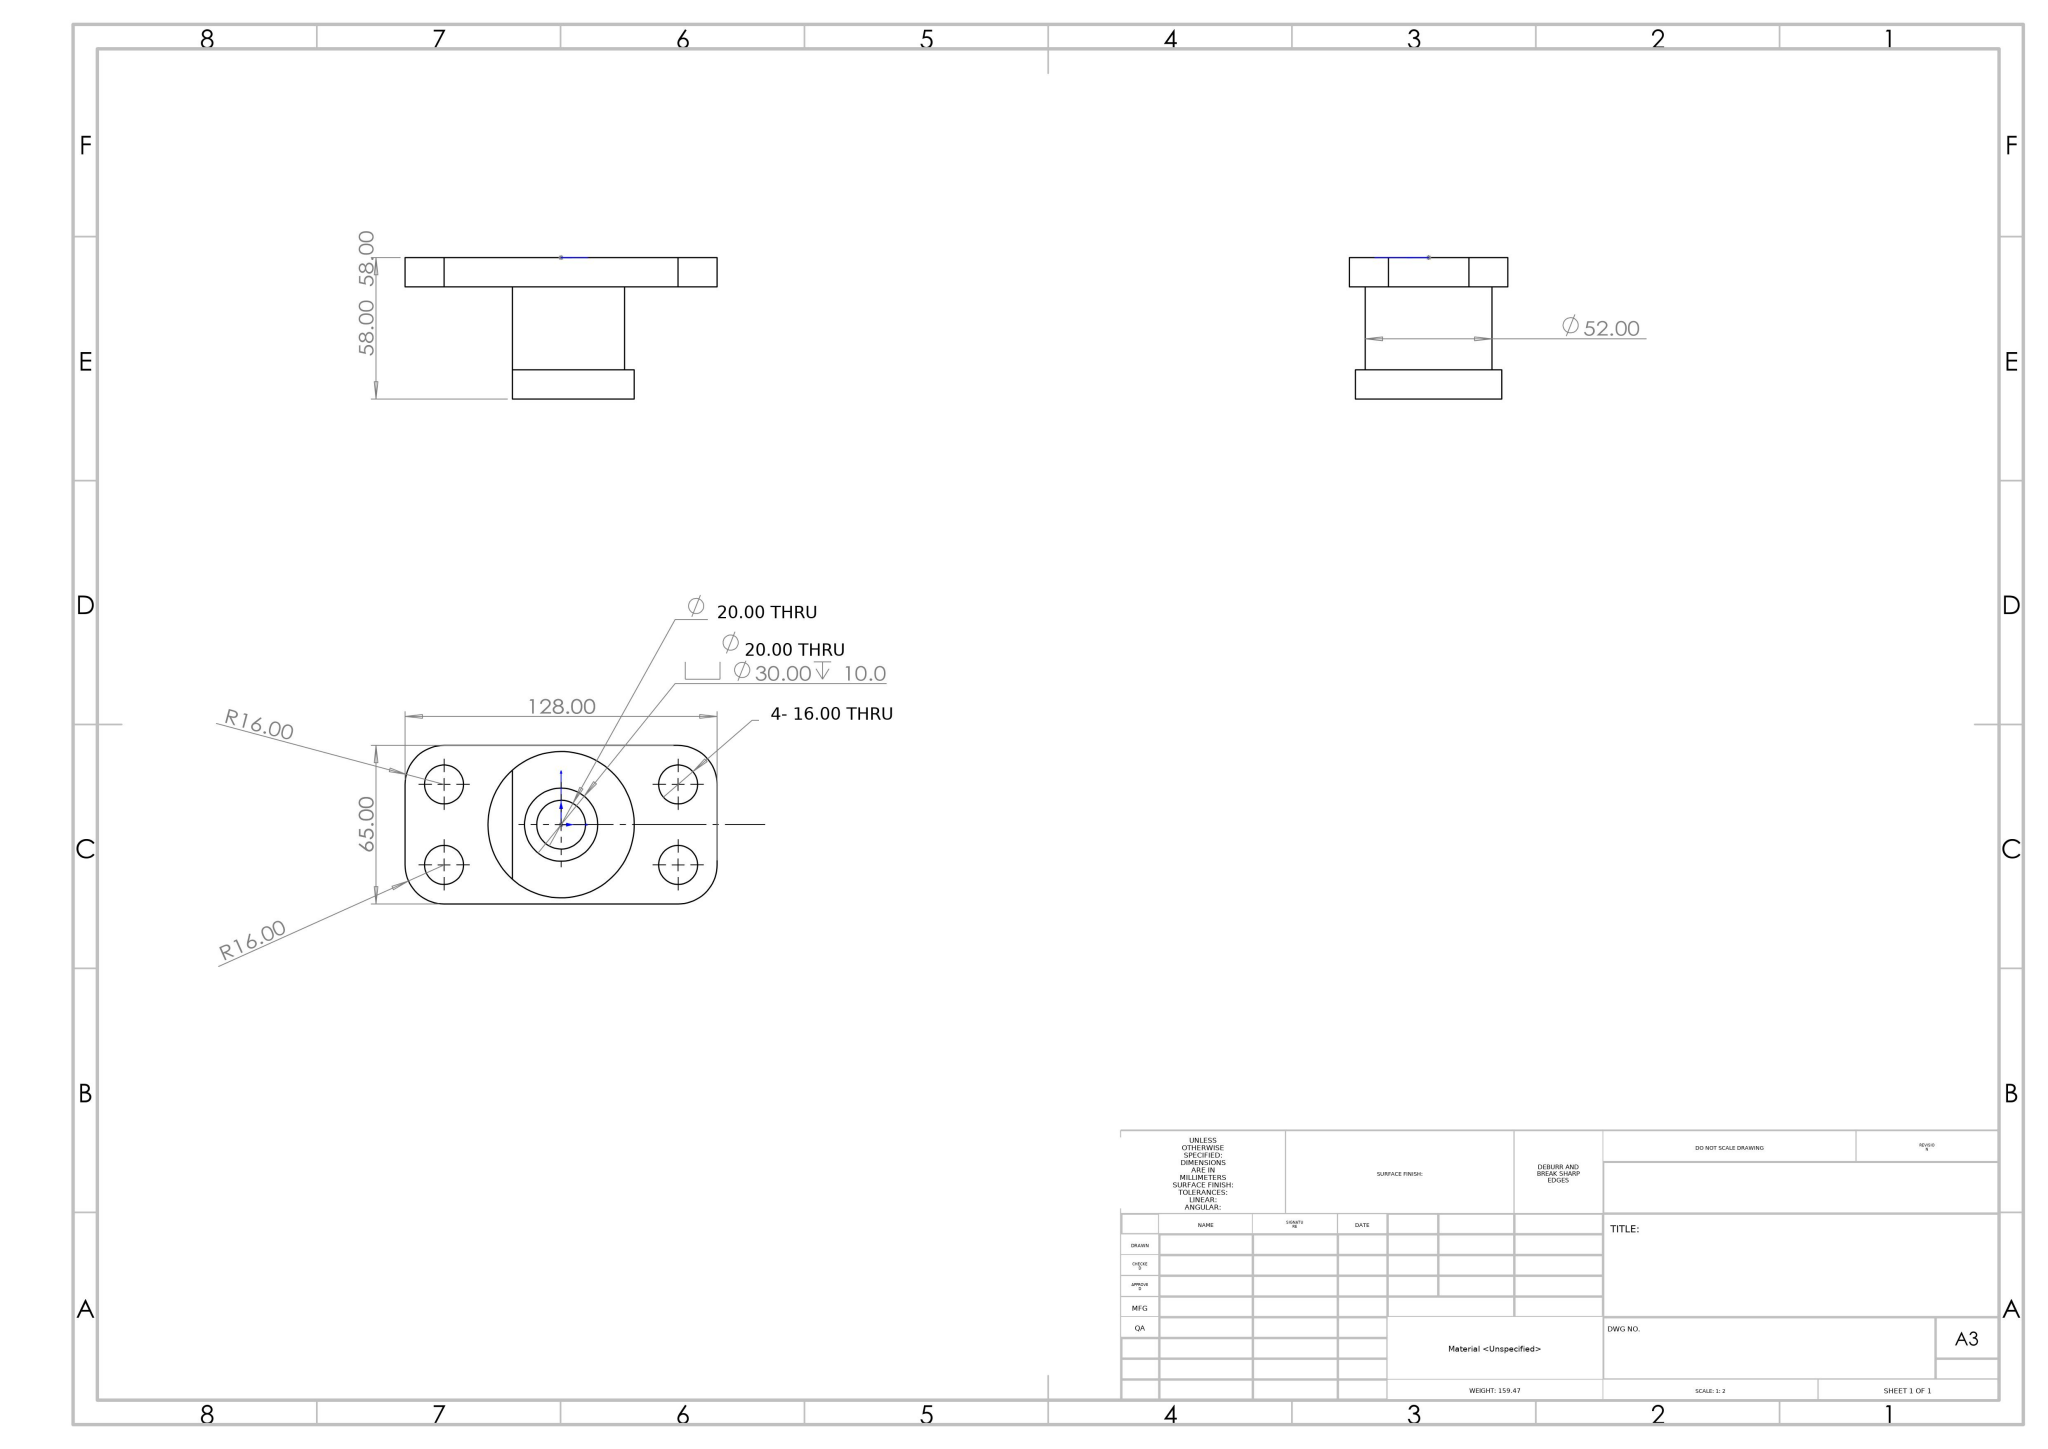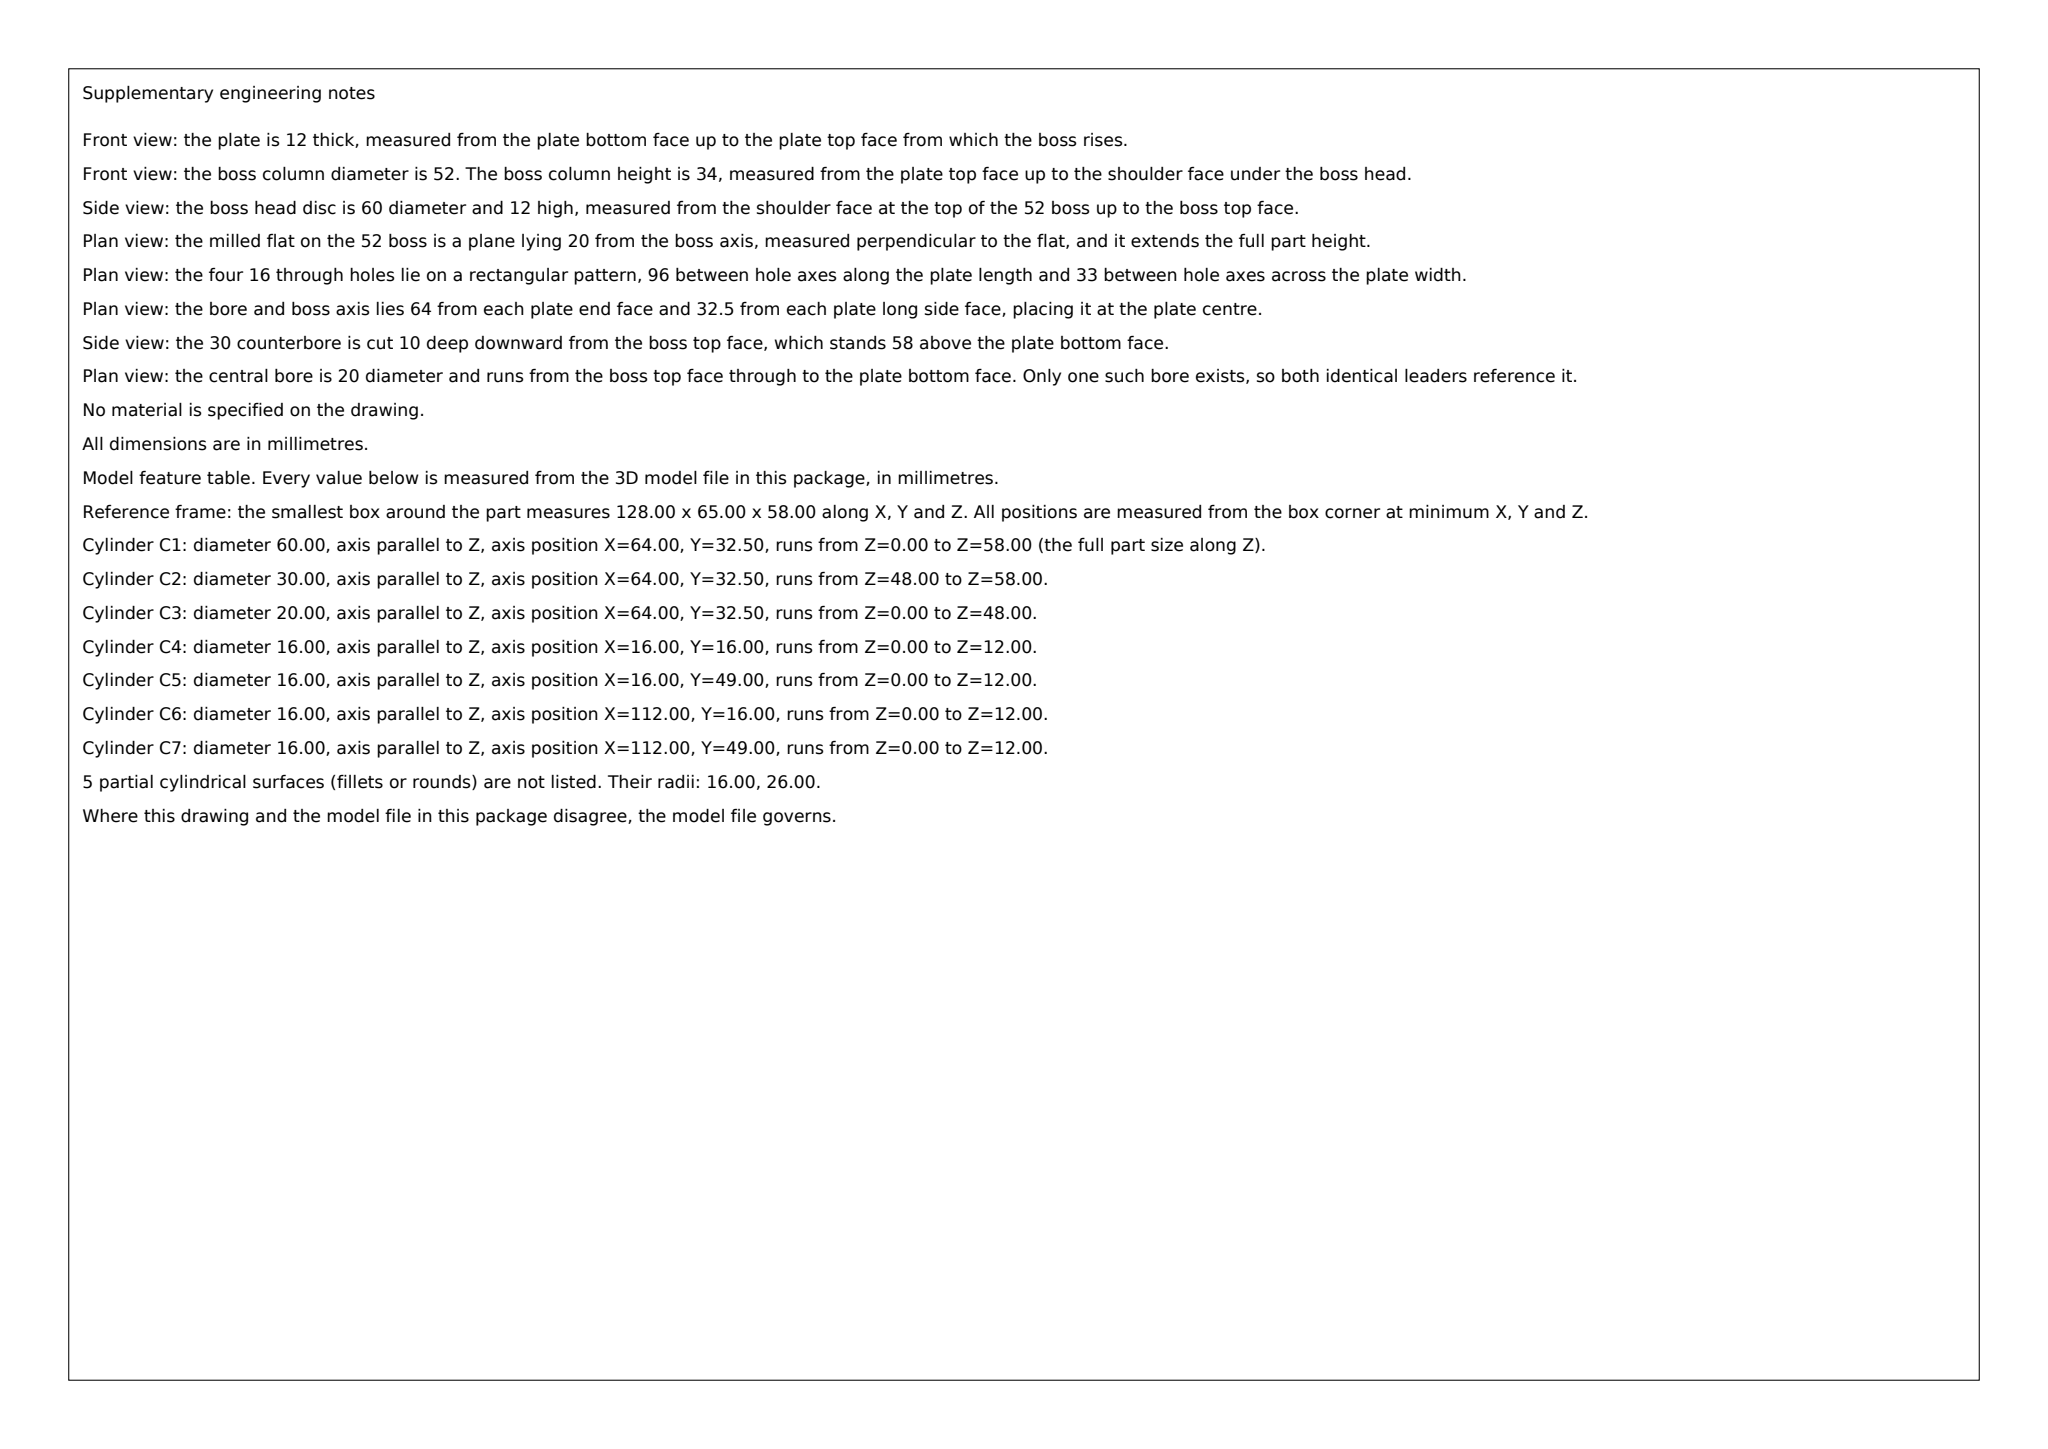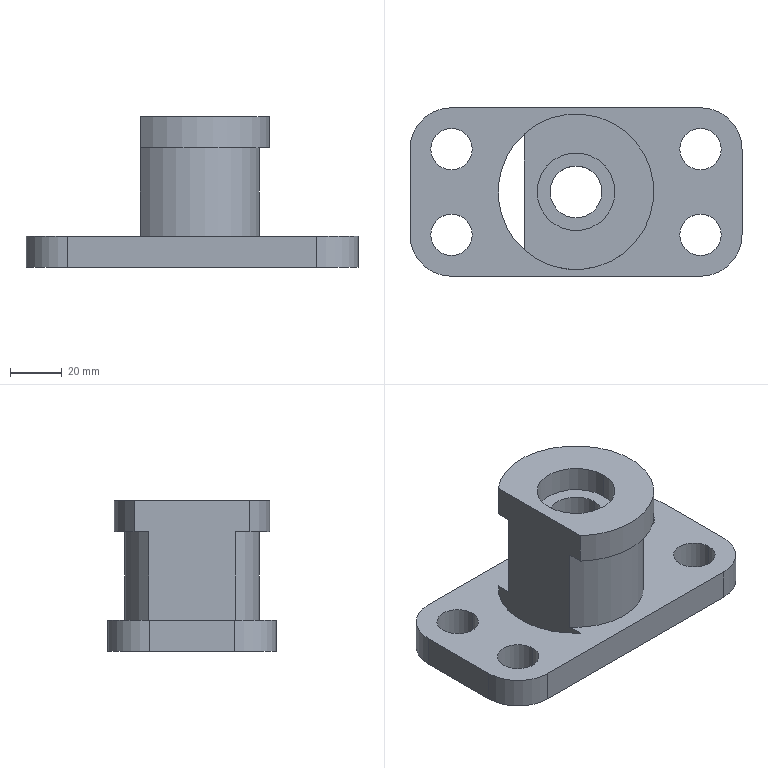Part | SolidWorks | mm | 1 solid | 29 faces | box 128 x 65 x 58 mm | volume 159471 mm3 | cylinder 19 | plane 10 | commonest cylinder face diameters 16 x8 32 x4 20 x2 30 x2 60 x2 52 x1
Drawing notes:
MILLED FLAT ON Ø60/Ø52 BOSS: 20 FROM BOSS AXIS, 44 FROM LH EDGE | from the solid: Plane normal x at x=44, extent y 10.1-54.9, z 0-58; boss axis at x=64,y=32.5
FLAT RUNS FULL 58 HT, PARALLEL TO 65.00 EDGE | from the solid: x=44 plane z range 0-58, normal along x (perp to 128.00 edge)
Ø60 SEGMENT NOTCH THRU 12 PLATE, FLAT AT 20 FROM BOSS AXIS | from the solid: Concave arc Ø60 at (64,32.5), z 0-12, 96 deg, bounded by x=44 plane
4-Ø16.00 THRU | from the solid: 4 bores Ø16 z 0-12 at (16,16),(112,16),(16,49),(112,49)
Ø20.00 THRU, CBORE Ø30.00 DP 10.0 FROM TOP FACE OF BOSS | from the solid: Bore Ø20 z 0-48; bore Ø30 z 48-58 (top face z=58)
build123d program:
from build123d import *

# Parameters (mm, degrees)
SKETCH1_W               = 128
SKETCH1_H               = 65
BOSS_EXTRUDE1_DEPTH     = 12
SKETCH2_R               = 26
BOSS_EXTRUDE2_DEPTH     = 34
SKETCH3_R               = 30
BOSS_EXTRUDE4_DEPTH     = 12
CUT_EXTRUDE1_REACH      = 94.284
SKETCH10_R              = 15
CUT_EXTRUDE2_DEPTH      = 10
SKETCH11_R              = 10
CUT_EXTRUDE3_DEPTH      = 87.35
SKETCH12_R              = 8
CUT_EXTRUDE5_DEPTH      = 86.254
MIRROR4_COPY_1_SKETCH_R = 8
MIRROR4_COPY_1_DEPTH    = 86.254
FILLET1_R               = 16


with BuildPart() as part:
    # Sketch1 → Boss-Extrude1 (new body)
    with BuildSketch(Plane.XY):
        Rectangle(SKETCH1_W, SKETCH1_H)
    extrude(amount=BOSS_EXTRUDE1_DEPTH)

    # Sketch2 → Boss-Extrude2 (add)
    with BuildSketch(Plane.XY.offset(12)):
        Circle(SKETCH2_R)
    extrude(amount=BOSS_EXTRUDE2_DEPTH)

    # Sketch3 → Boss-Extrude4 (add)
    with BuildSketch(Plane.XY.offset(46)):
        Circle(SKETCH3_R)
    extrude(amount=BOSS_EXTRUDE4_DEPTH)

    # Sketch7 → Cut-Extrude1 (cut, up to next)
    with BuildSketch(Plane.XY.offset(58), mode=Mode.PRIVATE) as cut_extrude1_sk1:
        with BuildLine():
            ThreePointArc((-20, 22.361), (-30, 0), (-20, -22.361))
            Line((-20, -22.361), (-20, 22.361))
        make_face()
    cut_extrude1_tool1 = extrude(cut_extrude1_sk1.sketch, amount=-CUT_EXTRUDE1_REACH, mode=Mode.PRIVATE) & part.part
    add(cut_extrude1_tool1.solids().sort_by_distance((-24.063, 0, 58))[0], mode=Mode.SUBTRACT)

    # Sketch10 → Cut-Extrude2 (cut)
    with BuildSketch(Plane.XY.offset(58)):
        Circle(SKETCH10_R)
    extrude(amount=-CUT_EXTRUDE2_DEPTH, mode=Mode.SUBTRACT)

    # Sketch11 → Cut-Extrude3 (cut, through all)
    with BuildSketch(Plane.XY.offset(48)):
        Circle(SKETCH11_R)
    extrude(amount=-CUT_EXTRUDE3_DEPTH, mode=Mode.SUBTRACT)

    # Sketch12 → Cut-Extrude5 (cut, through all)
    with BuildSketch(Plane.XY.offset(12)):
        with Locations((-48, -16.5)):
            Circle(SKETCH12_R)
    cut_extrude5 = extrude(amount=-CUT_EXTRUDE5_DEPTH, mode=Mode.SUBTRACT)

    # Mirror2: Cut-Extrude5 across plane
    add(cut_extrude5.mirror(Plane.XY), mode=Mode.SUBTRACT)

    # Mirror3: Cut-Extrude5 across plane
    add(cut_extrude5.mirror(Plane(origin=(0, 0, 0), x_dir=(0, 0, 1), z_dir=(1, 0, 0))), mode=Mode.SUBTRACT)

    # Mirror4: Cut-Extrude5 across plane
    add(cut_extrude5.mirror(Plane.ZX), mode=Mode.SUBTRACT)

    # Mirror4 copy 1 sketch → Mirror4 copy 1 (cut, through all)
    with BuildSketch(Plane(origin=(0, 0, 12), x_dir=(-1, 0, 0), z_dir=(0, 0, 1))):
        with Locations((-48, -16.5)):
            Circle(MIRROR4_COPY_1_SKETCH_R)
    extrude(amount=-MIRROR4_COPY_1_DEPTH, mode=Mode.SUBTRACT)

    # Fillet1
    fillet1_edges = [part.edges().sort_by_distance(p)[0] for p in [
        (64, -32.5, 6),
        (-64, -32.5, 6),
        (-64, 32.5, 6),
        (64, 32.5, 6),
    ]]
    fillet(fillet1_edges, radius=FILLET1_R)


solid = part.part